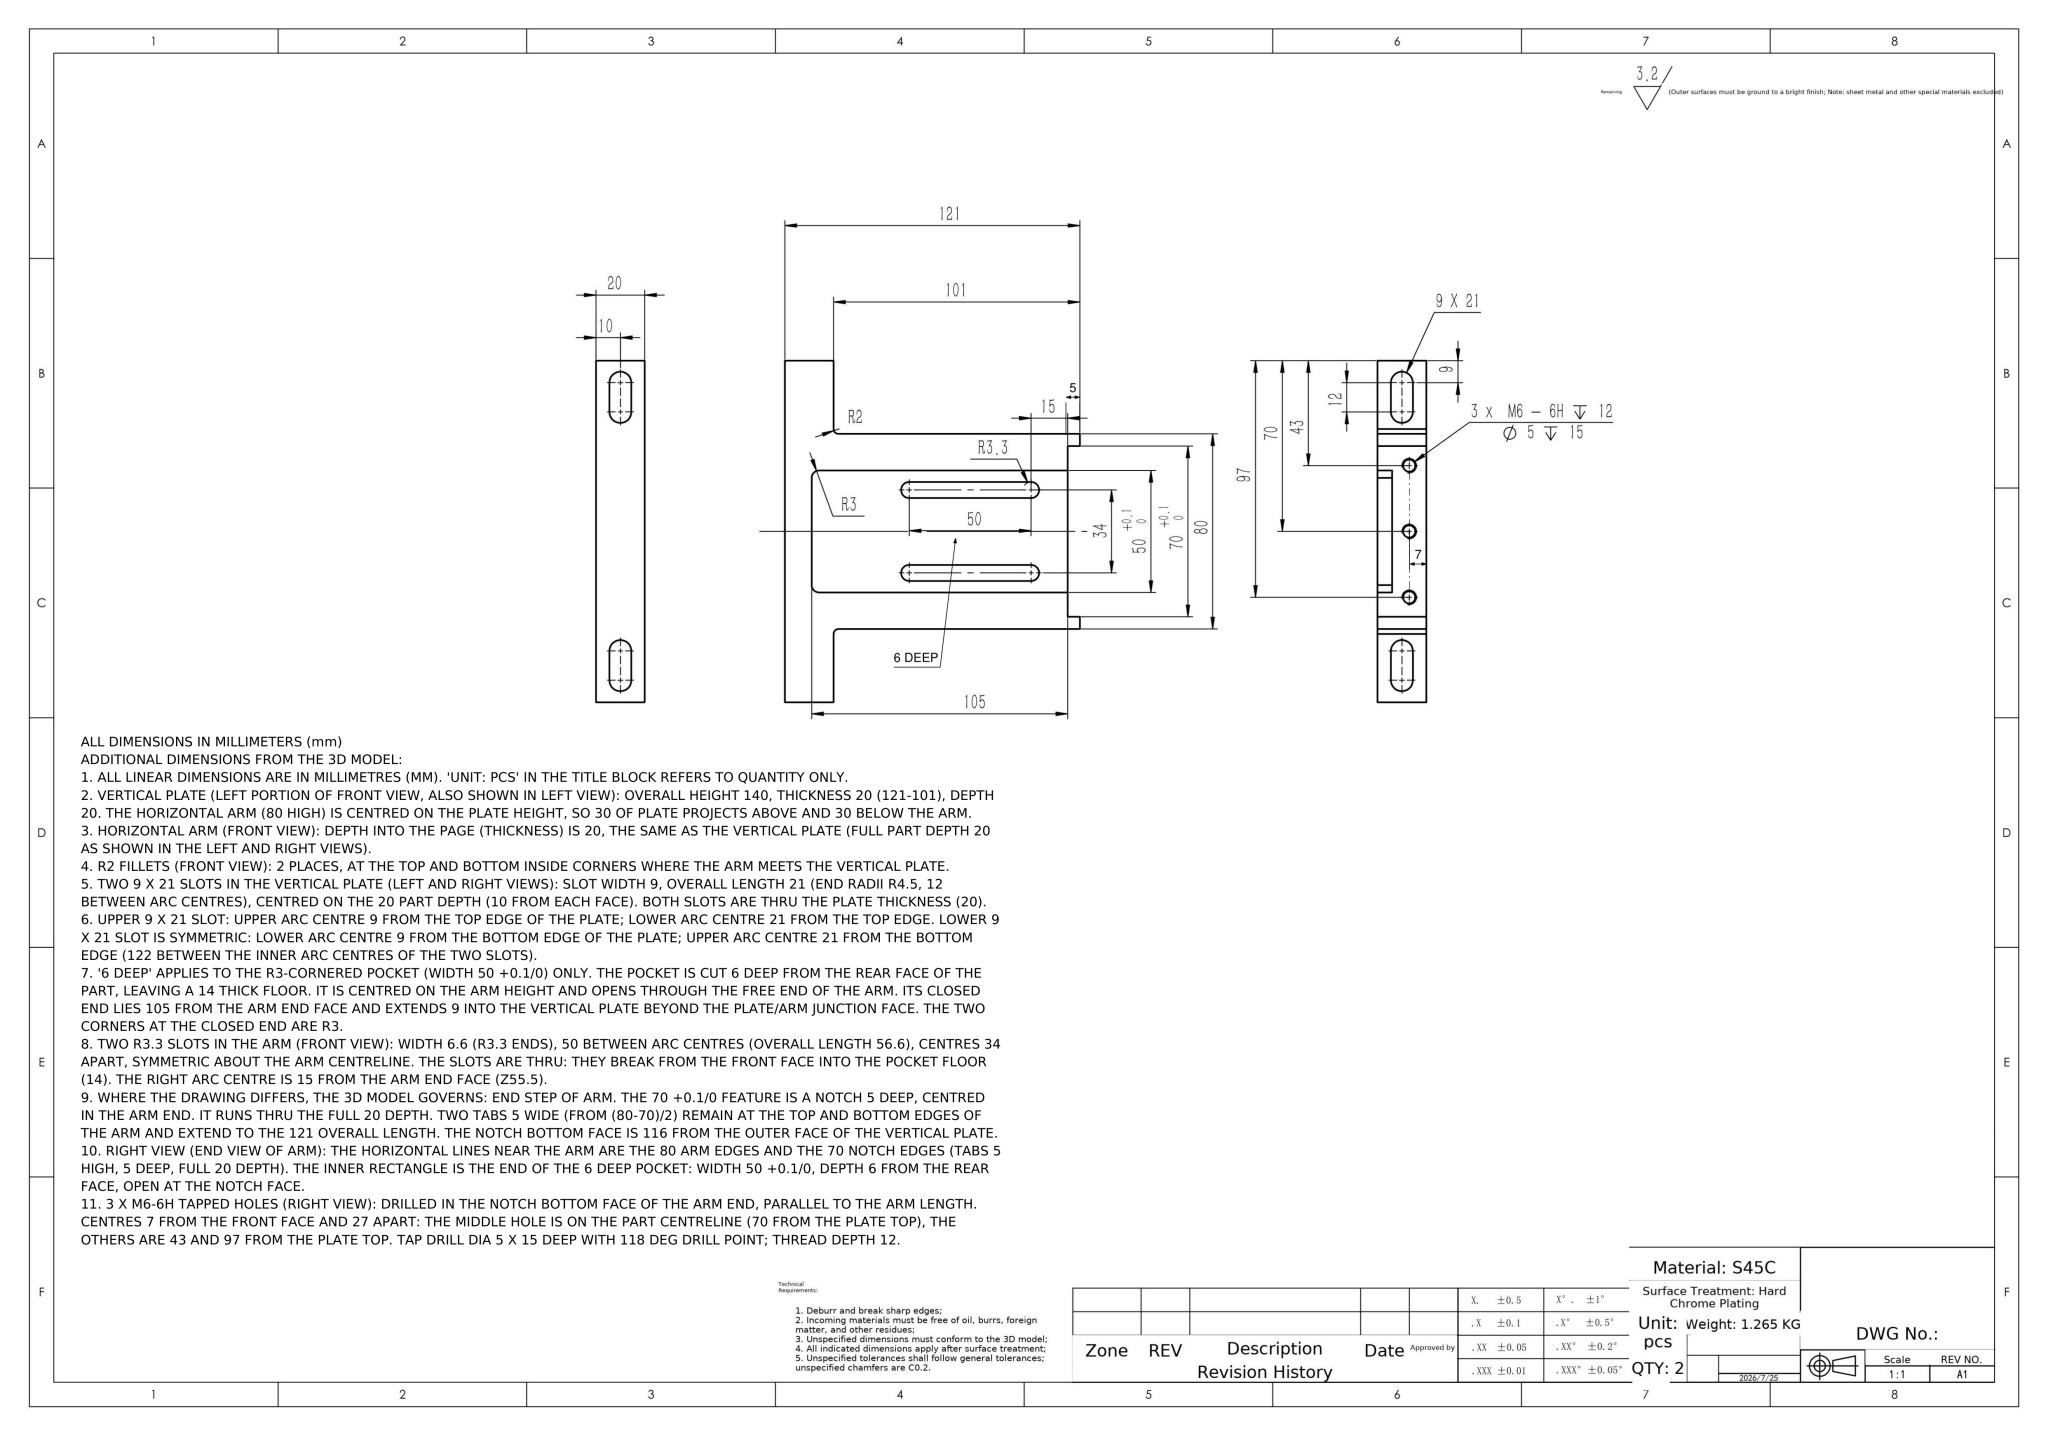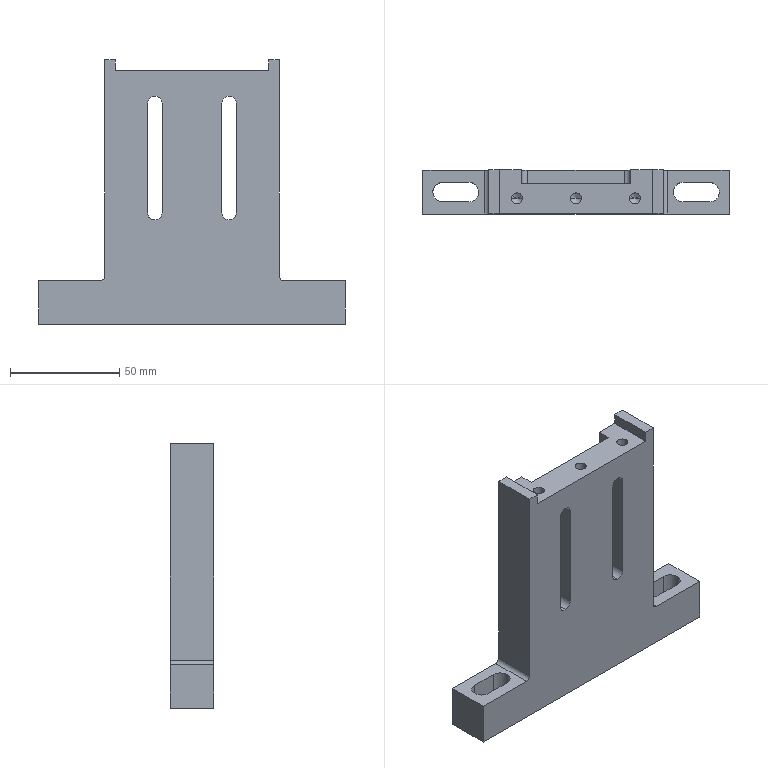Part | NX | mm | L-Shaped Slotted Motor Bracket | 1 solid | 54 faces | box 140 x 20 x 121 mm | volume 161182 mm3 | plane 26 | cylinder 22 | cone 6 | commonest cylinder face diameters 9 x6 6.6 x6 5 x6 4 x2 6 x2